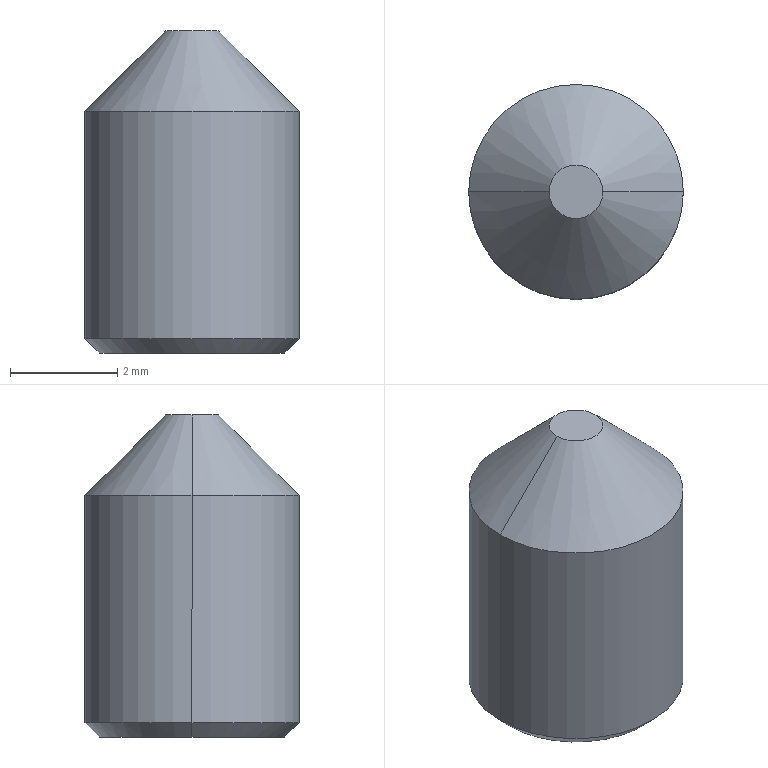Component | SolidWorks | LiftingPlateAssembly-1_GB_T78-2000HexagonSocketConePointSetScrewM4x6-1 | 1 solid | 22 faces | box 4 x 4 x 6 mm | volume 59 mm3 | plane 14 | cone 6 | cylinder 2 | commonest cylinder face diameters 4 x2
build123d program:
from build123d import *

# Parameters (mm, degrees)
CUT_EXTRUDE1_DEPTH = 1.5


with BuildPart() as part:
    # Sketch1 → Base-Revolve (revolve)
    with BuildSketch(Plane.XY, mode=Mode.PRIVATE) as base_revolve_sk:
        Polygon((0, 0), (6, 0), (6, 0.5), (4.5, 2), (0.268, 2), (0, 1.732), align=None)
    revolve(base_revolve_sk.sketch.rotate(Axis((-1.41, 0, 0), (1, 0, 0)), 90), axis=Axis((-1.41, 0, 0), (1, 0, 0)))

    # Sketch2 → Cut-Extrude1 (cut)
    with BuildSketch(Plane.ZY):
        Polygon((1.15, 0), (0.575, 0.9959), (-0.575, 0.9959), (-1.15, 0), (-0.575, -0.9959), (0.575, -0.9959), align=None)
    extrude(amount=-CUT_EXTRUDE1_DEPTH, mode=Mode.SUBTRACT)

    # Sketch3 → Cut-Revolve1 (revolve, cut)
    with BuildSketch(Plane.XY, mode=Mode.PRIVATE) as cut_revolve1_sk:
        Polygon((1.5, 0.9959), (2.075, 0), (1.5, 0), align=None)
    revolve(cut_revolve1_sk.sketch.rotate(Axis((-0.1213, 0, 0), (1, 0, 0)), 90), axis=Axis((-0.1213, 0, 0), (1, 0, 0)), mode=Mode.SUBTRACT)


solid = part.part

# Placed as in the assembly
solid = solid.moved(Location((-212.5, 2, -76), (0, -90, 0)))